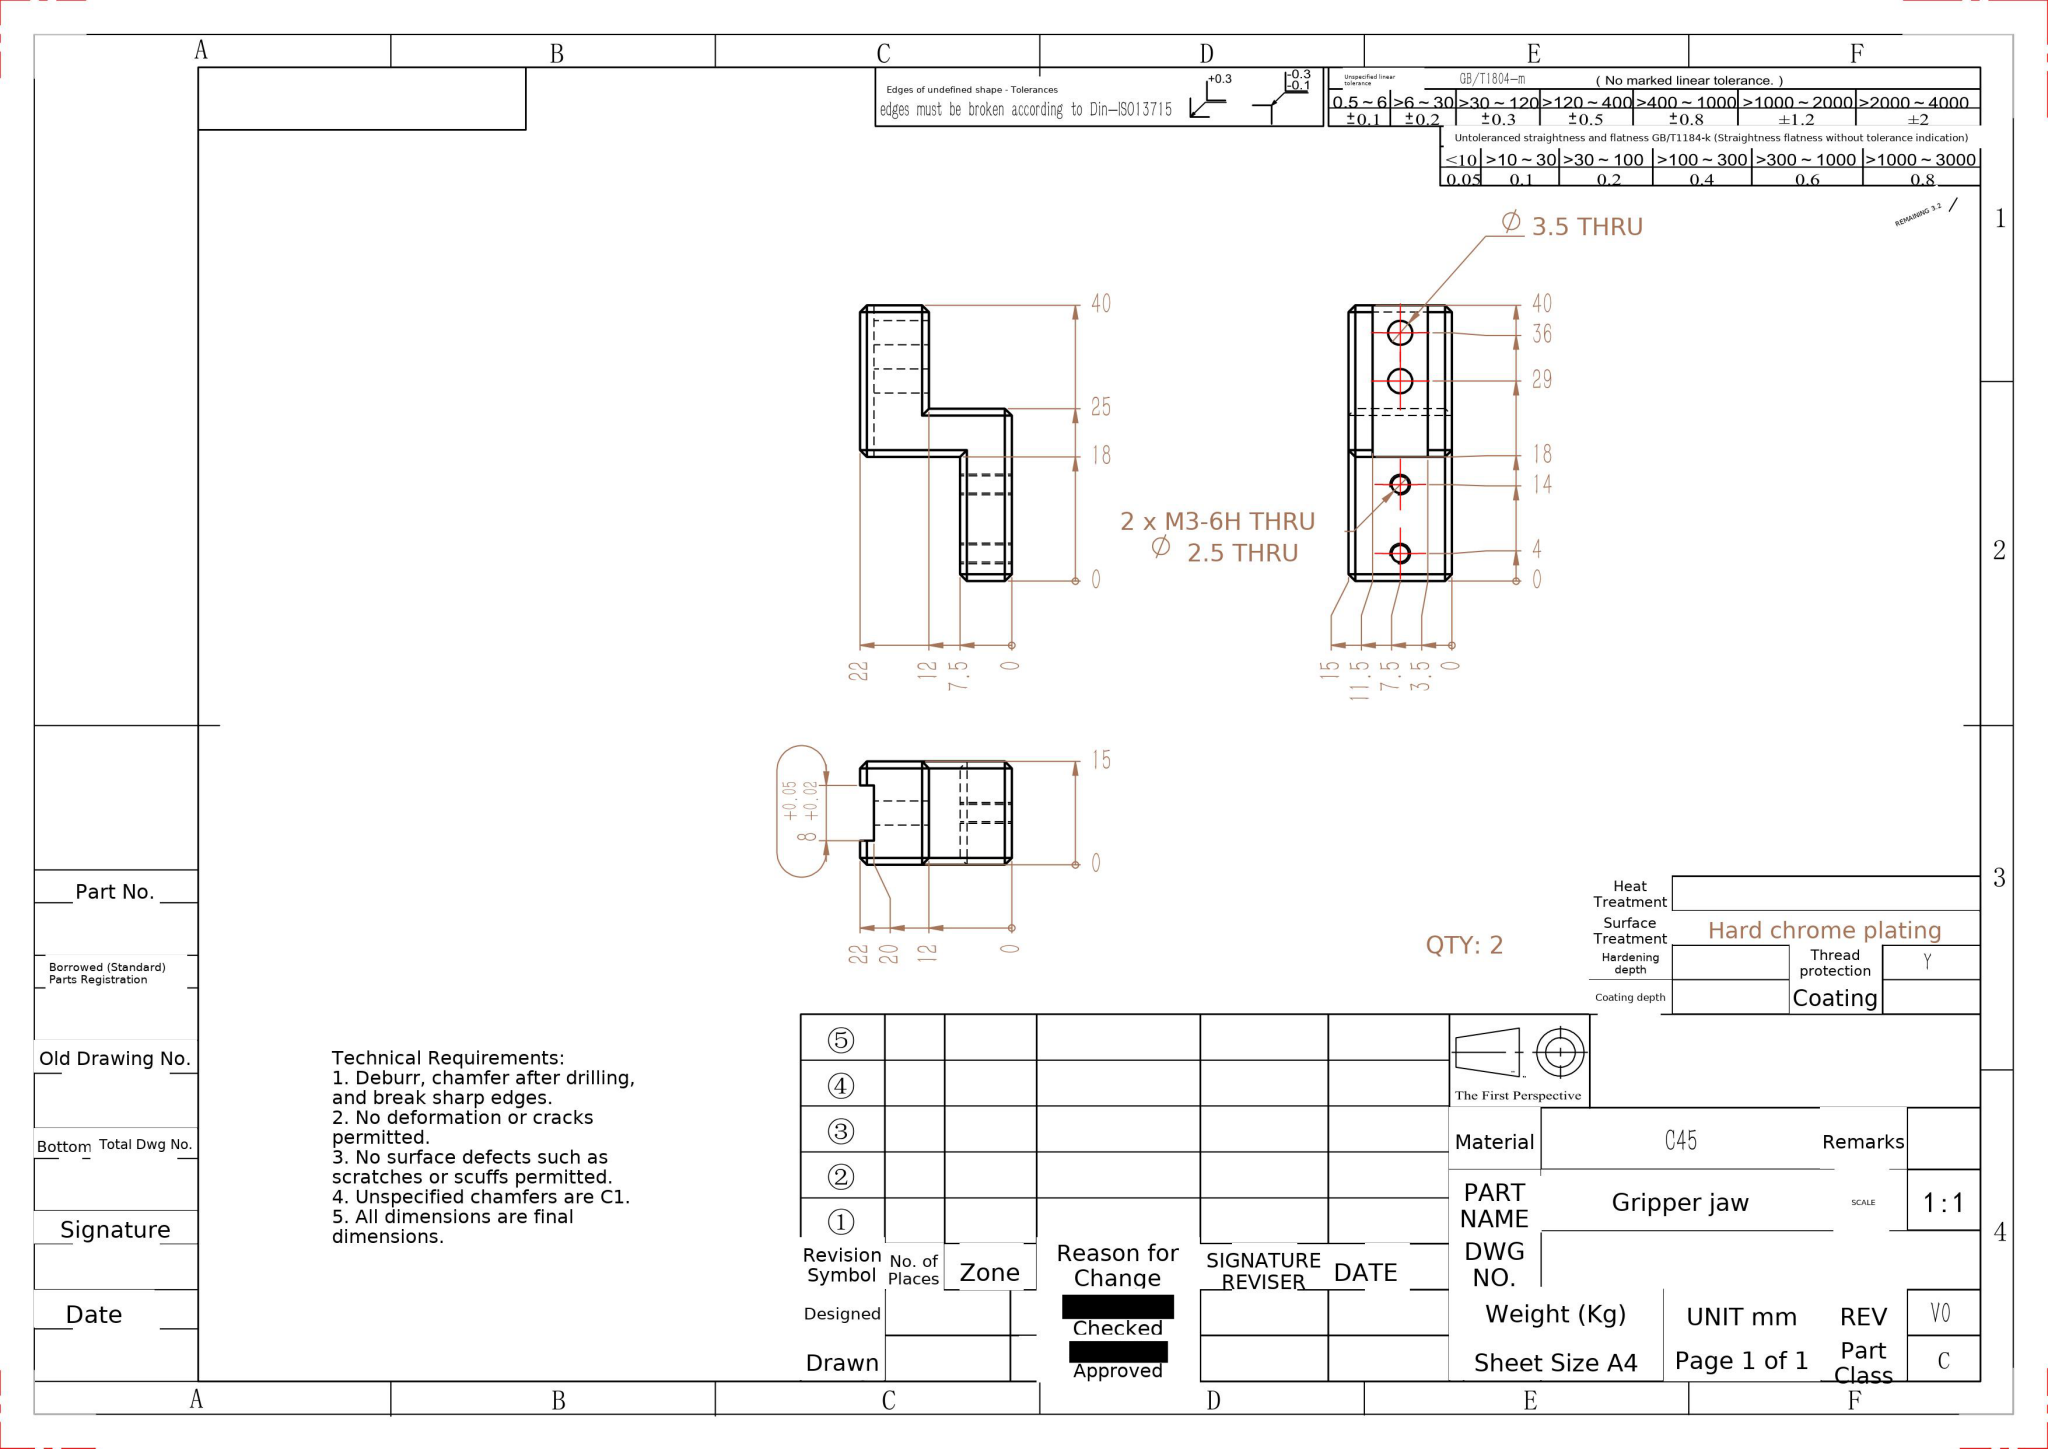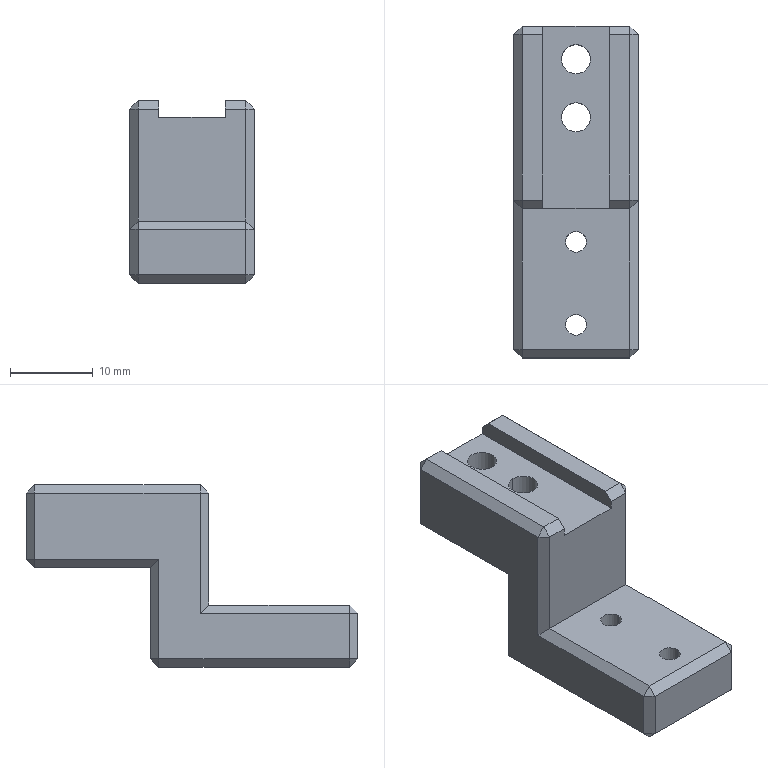Part | NX | mm | 1 solid | 58 faces | box 15 x 40 x 22 mm | volume 5851 mm3 | plane 50 | cylinder 8 | commonest cylinder face diameters 2.5 x4 3.5 x4